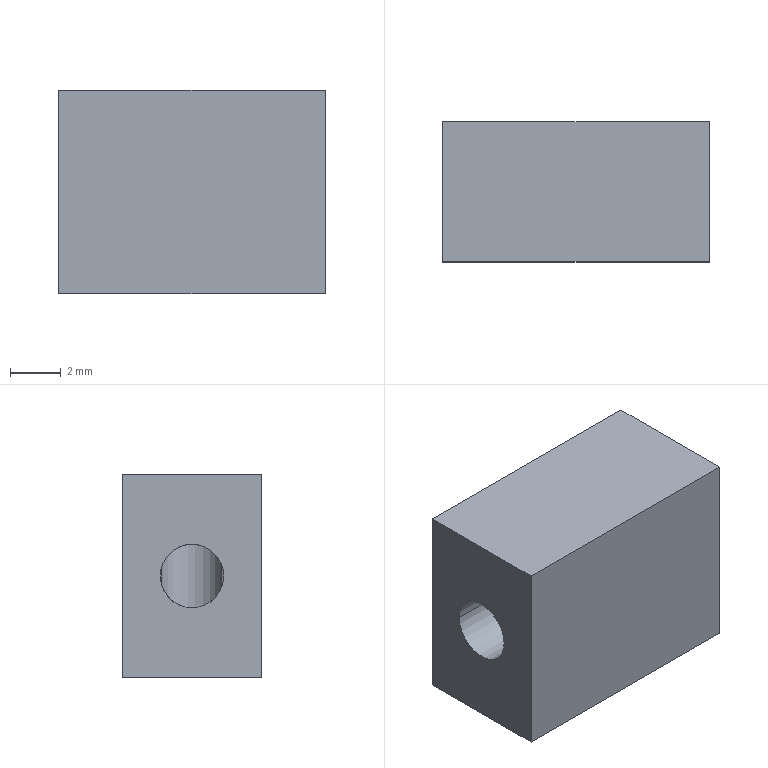CAM job | Mastercam | mm | 8 operations | part box 10.5 x 5.5 x 8
1. Facing | 24 - 100 平铣刀
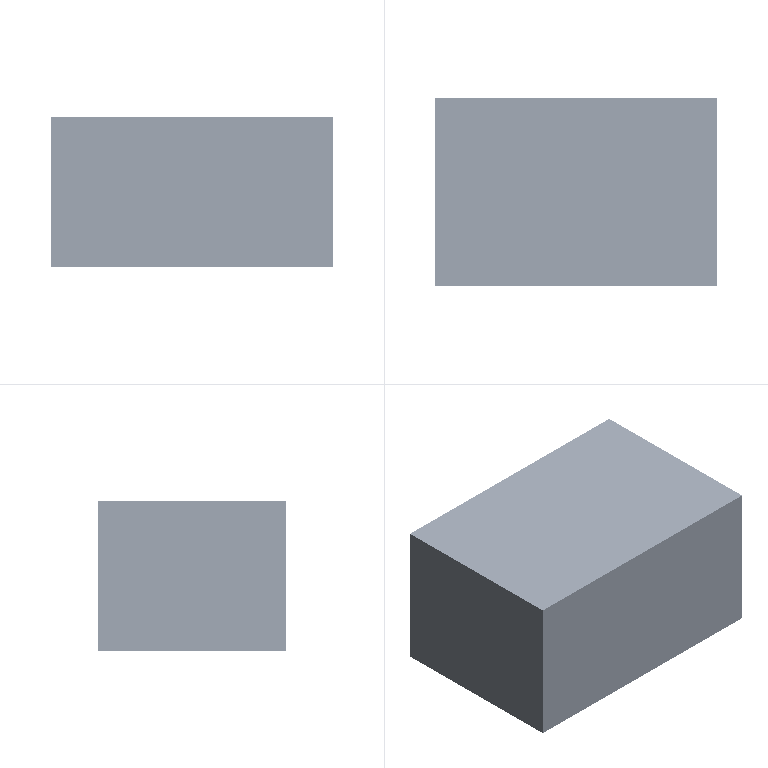2. Contour (Ramp) | 9 - 10 平铣刀
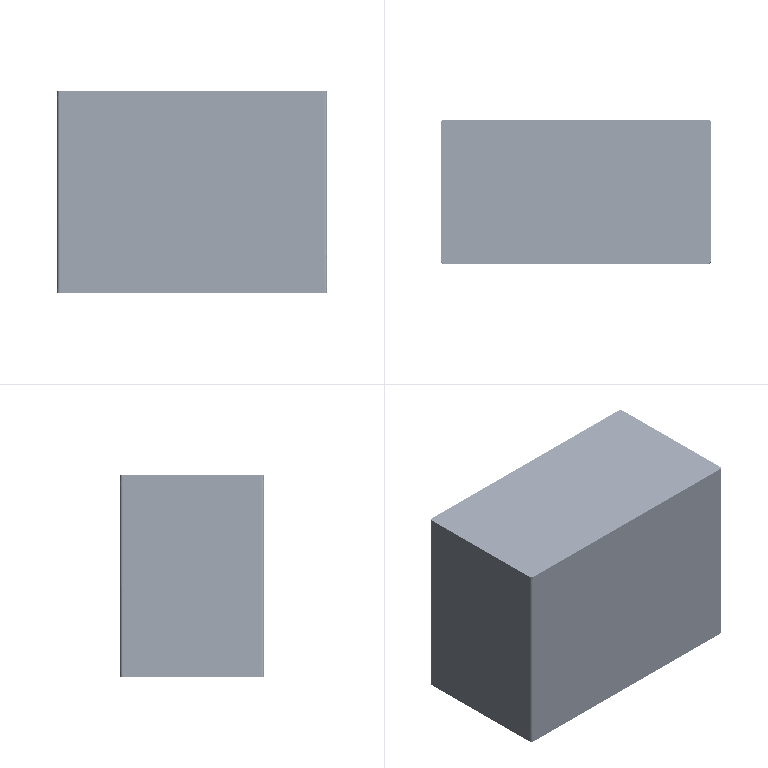3. Contour (2D) | 10 - 10 平铣刀
4. Drill/Counterbore | 5 - 4 倒角刀
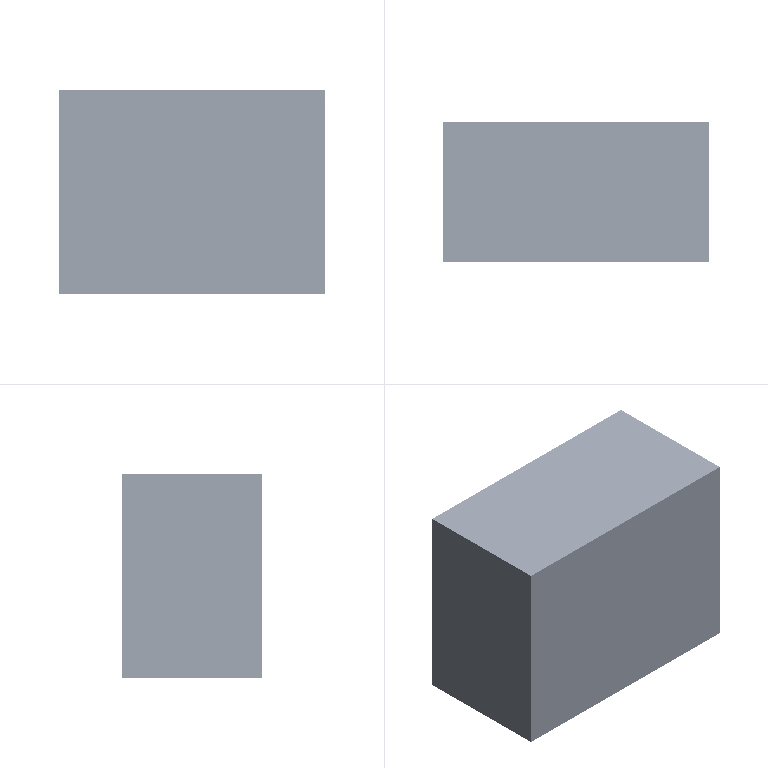5. Contour (2D chamfer) | 5 - 4 倒角刀
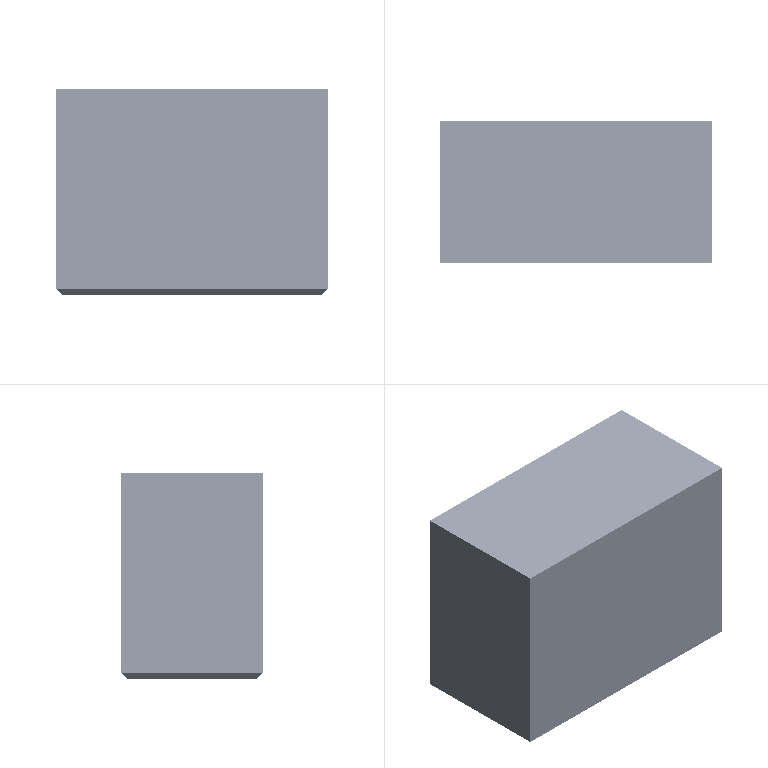6. Facing | 24 - 100 平铣刀
7. Contour (2D chamfer) | 5 - 4 倒角刀
8. Drill/Counterbore | 5 - 4 倒角刀